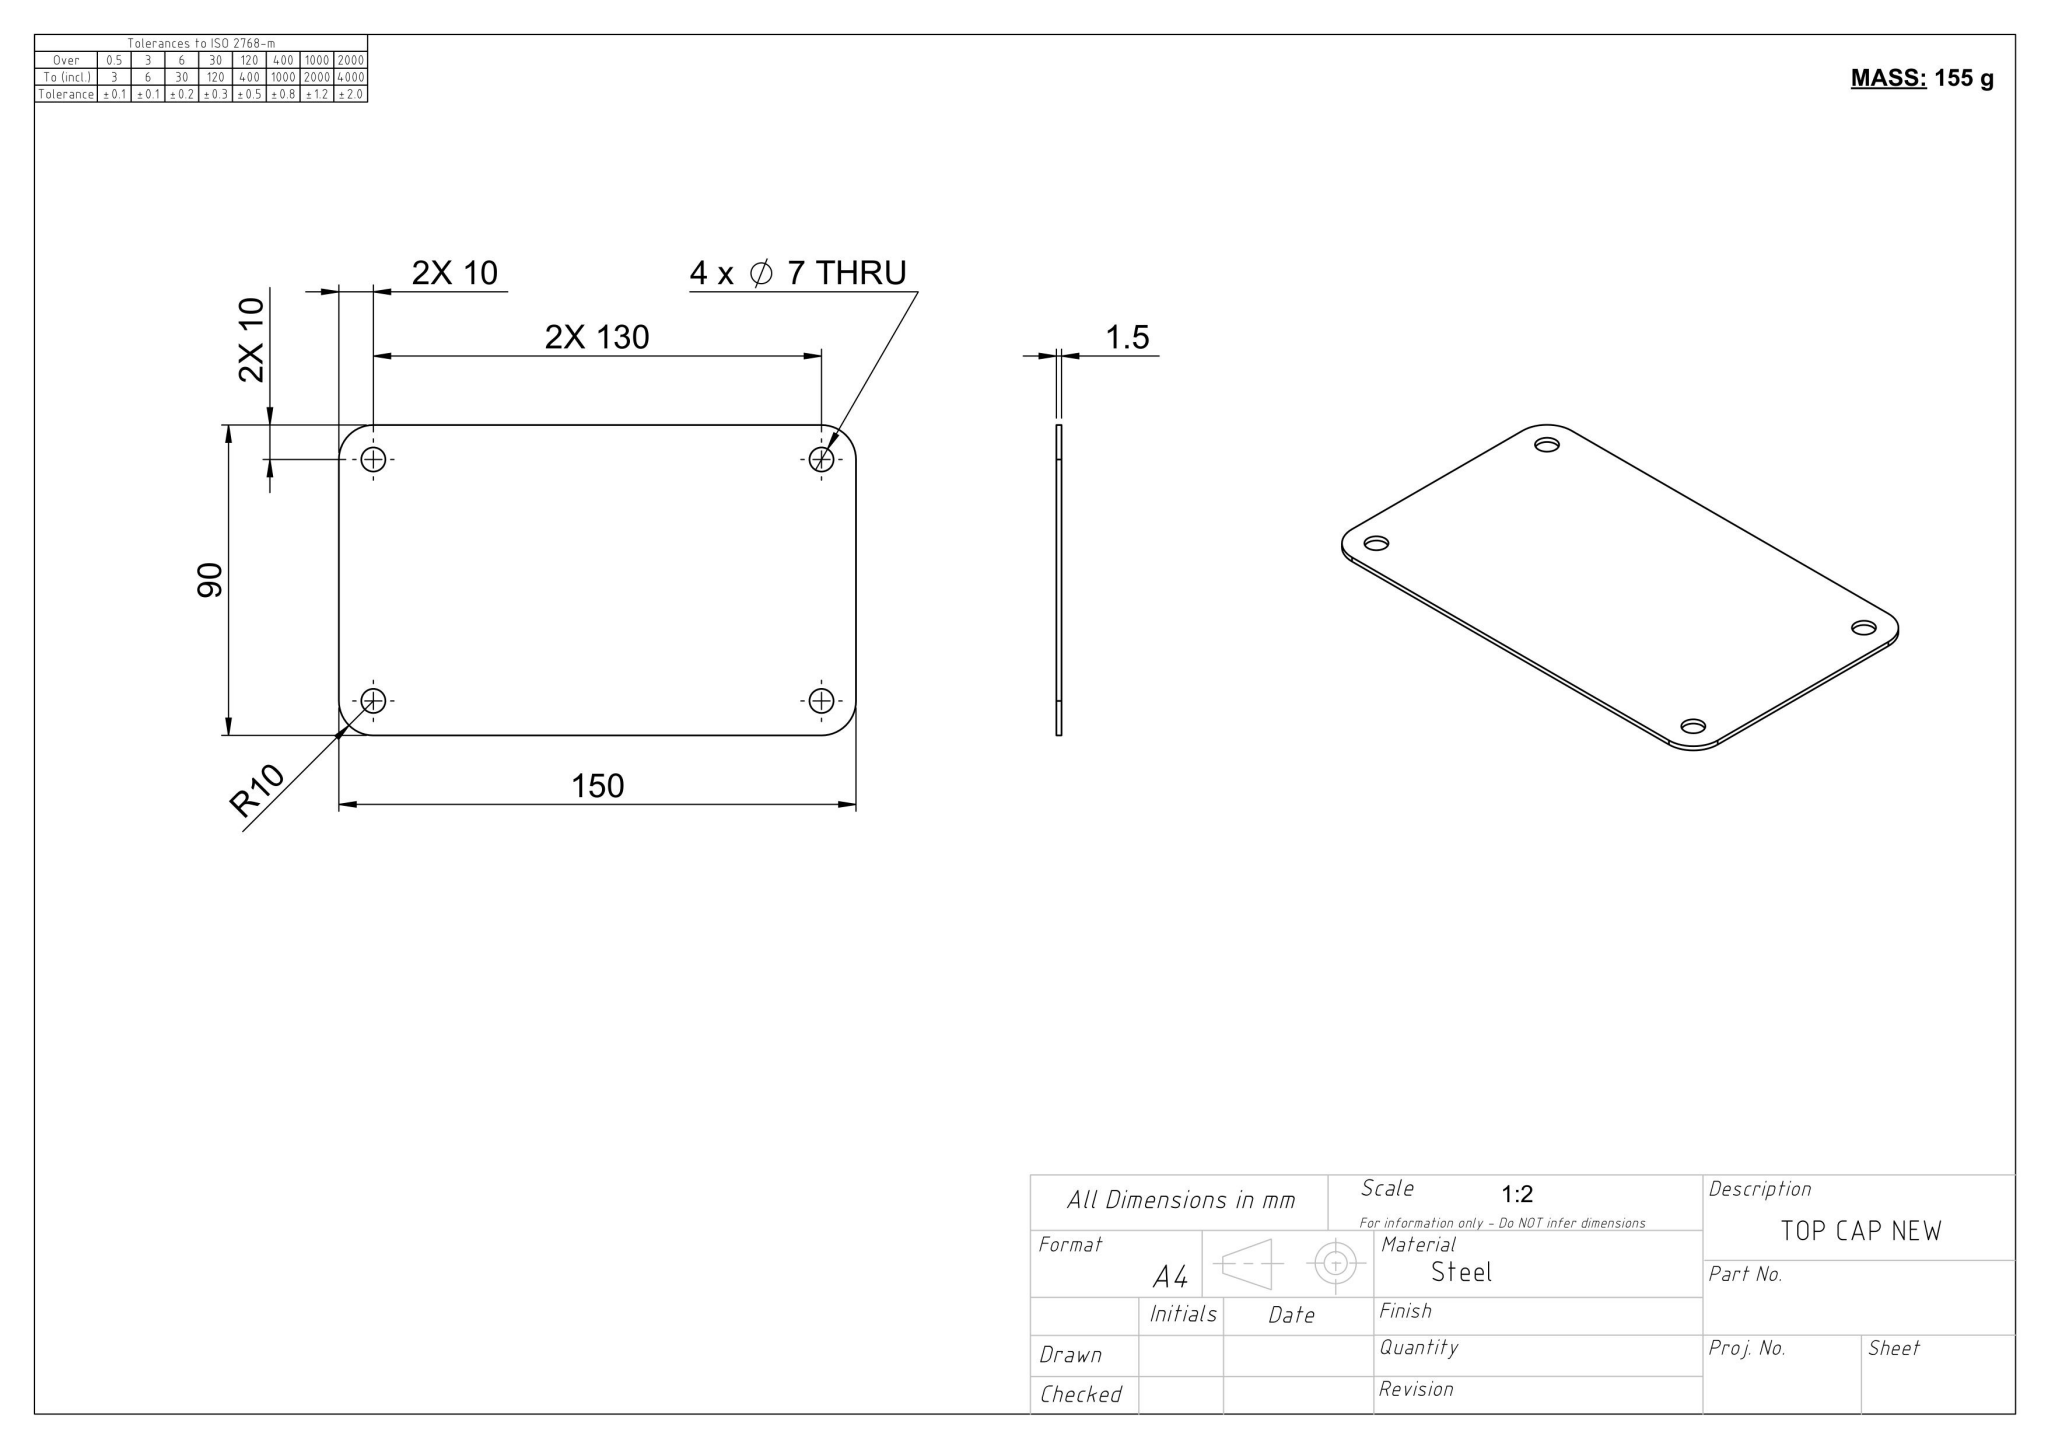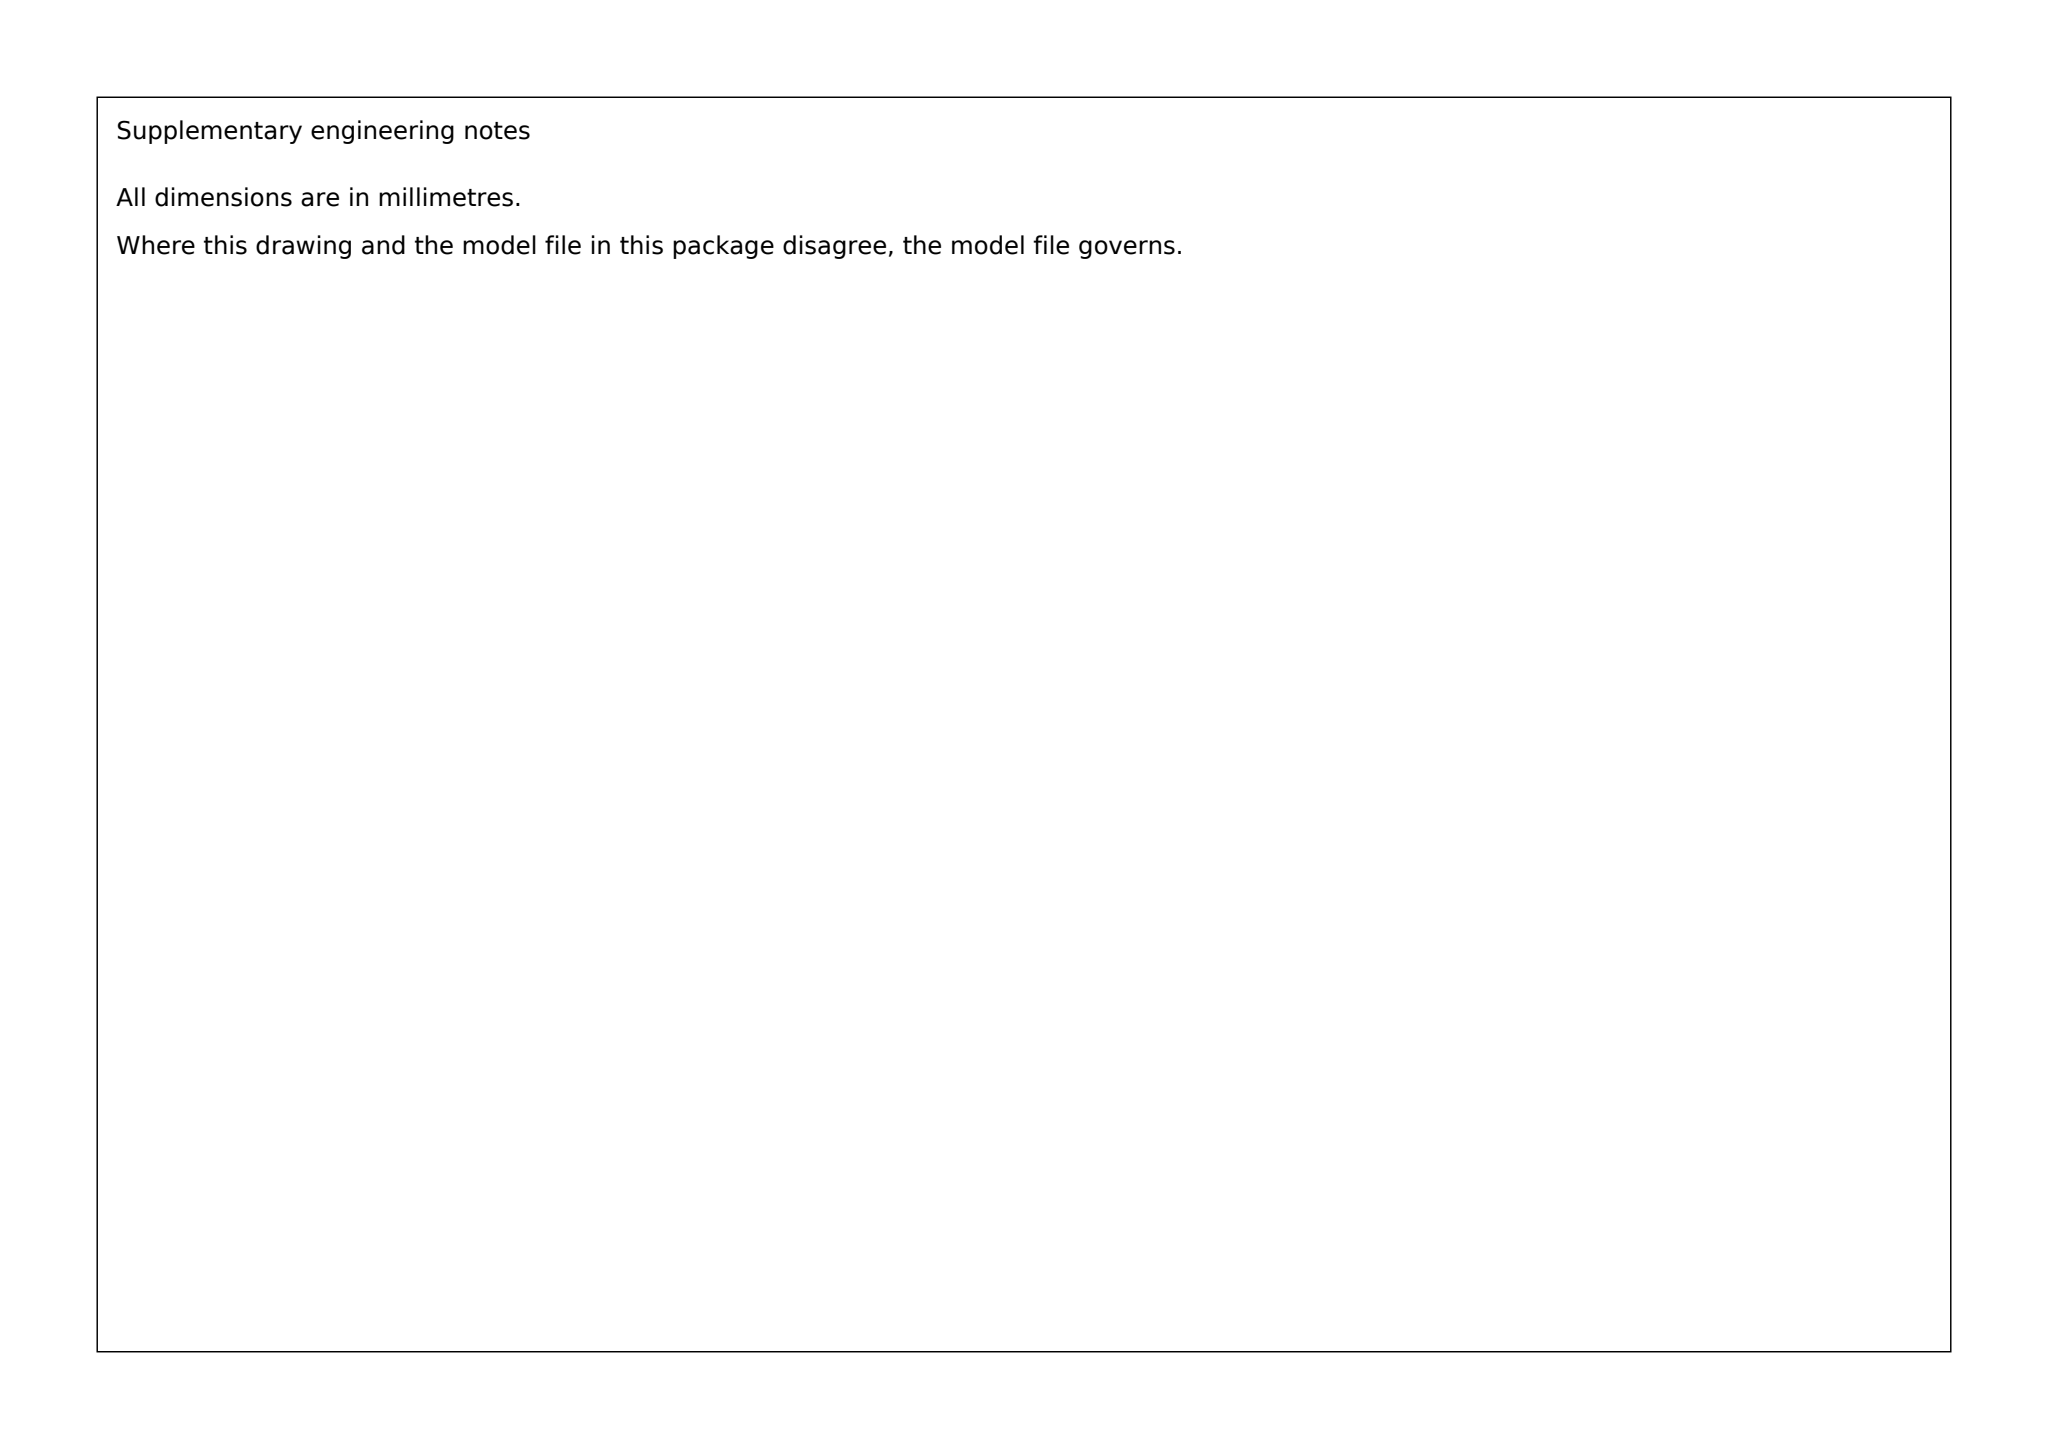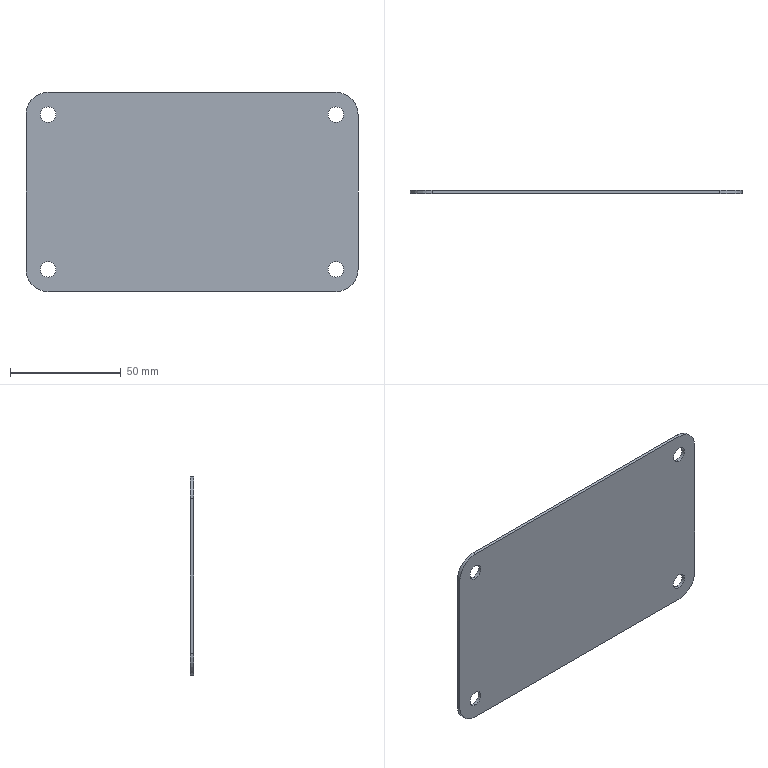Part | SolidWorks | mm | material Steel | 1 solid | 18 faces | box 150 x 1.5 x 90 mm | volume 19890 mm3 | cylinder 12 | plane 6 | commonest cylinder face diameters 7 x8 20 x4
STEP:
#1=CARTESIAN_POINT('',(-65.,0.,-38.5));
#2=VERTEX_POINT('',#1);
#3=CARTESIAN_POINT('',(-65.,0.,-31.5));
#4=VERTEX_POINT('',#3);
#5=CARTESIAN_POINT('',(-65.,0.,-35.));
#6=DIRECTION('',(0.,1.,0.));
#7=DIRECTION('',(0.,0.,1.));
#8=AXIS2_PLACEMENT_3D('',#5,#6,#7);
#9=CIRCLE('',#8,3.5);
#10=EDGE_CURVE('',#2,#4,#9,.T.);
#11=ORIENTED_EDGE('',*,*,#10,.F.);
#12=CARTESIAN_POINT('',(-65.,1.5,-38.5));
#13=VERTEX_POINT('',#12);
#14=CARTESIAN_POINT('',(-65.,1.5,-38.5));
#15=DIRECTION('',(0.,1.,0.));
#16=VECTOR('',#15,1000.);
#17=LINE('',#14,#16);
#18=EDGE_CURVE('',#2,#13,#17,.T.);
#19=ORIENTED_EDGE('',*,*,#18,.T.);
#20=CARTESIAN_POINT('',(-65.,1.5,-31.5));
#21=VERTEX_POINT('',#20);
#22=CARTESIAN_POINT('',(-65.,1.5,-35.));
#23=DIRECTION('',(0.,1.,0.));
#24=DIRECTION('',(0.,0.,1.));
#25=AXIS2_PLACEMENT_3D('',#22,#23,#24);
#26=CIRCLE('',#25,3.5);
#27=EDGE_CURVE('',#13,#21,#26,.T.);
#28=ORIENTED_EDGE('',*,*,#27,.T.);
#29=CARTESIAN_POINT('',(-65.,1.5,-31.5));
#30=DIRECTION('',(0.,1.,0.));
#31=VECTOR('',#30,1000.);
#32=LINE('',#29,#31);
#33=EDGE_CURVE('',#4,#21,#32,.T.);
#34=ORIENTED_EDGE('',*,*,#33,.F.);
#35=EDGE_LOOP('',(#11,#19,#28,#34));
#36=FACE_OUTER_BOUND('',#35,.T.);
#37=CARTESIAN_POINT('',(-65.,1.5,-35.));
#38=DIRECTION('',(0.,1.,0.));
#39=DIRECTION('',(0.,0.,1.));
#40=AXIS2_PLACEMENT_3D('',#37,#38,#39);
#41=CYLINDRICAL_SURFACE('',#40,3.5);
#42=ADVANCED_FACE('',(#36),#41,.F.);
#43=CARTESIAN_POINT('',(65.,0.,-38.5));
#44=VERTEX_POINT('',#43);
#45=CARTESIAN_POINT('',(65.,0.,-31.5));
#46=VERTEX_POINT('',#45);
#47=CARTESIAN_POINT('',(65.,0.,-35.));
#48=DIRECTION('',(0.,1.,0.));
#49=DIRECTION('',(0.,0.,1.));
#50=AXIS2_PLACEMENT_3D('',#47,#48,#49);
#51=CIRCLE('',#50,3.5);
#52=EDGE_CURVE('',#44,#46,#51,.T.);
#53=ORIENTED_EDGE('',*,*,#52,.F.);
#54=CARTESIAN_POINT('',(65.,1.5,-38.5));
#55=VERTEX_POINT('',#54);
#56=CARTESIAN_POINT('',(65.,1.5,-38.5));
#57=DIRECTION('',(0.,1.,0.));
#58=VECTOR('',#57,1000.);
#59=LINE('',#56,#58);
#60=EDGE_CURVE('',#44,#55,#59,.T.);
#61=ORIENTED_EDGE('',*,*,#60,.T.);
#62=CARTESIAN_POINT('',(65.,1.5,-31.5));
#63=VERTEX_POINT('',#62);
#64=CARTESIAN_POINT('',(65.,1.5,-35.));
#65=DIRECTION('',(0.,1.,0.));
#66=DIRECTION('',(0.,0.,1.));
#67=AXIS2_PLACEMENT_3D('',#64,#65,#66);
#68=CIRCLE('',#67,3.5);
#69=EDGE_CURVE('',#55,#63,#68,.T.);
#70=ORIENTED_EDGE('',*,*,#69,.T.);
#71=CARTESIAN_POINT('',(65.,1.5,-31.5));
#72=DIRECTION('',(0.,1.,0.));
#73=VECTOR('',#72,1000.);
#74=LINE('',#71,#73);
#75=EDGE_CURVE('',#46,#63,#74,.T.);
#76=ORIENTED_EDGE('',*,*,#75,.F.);
#77=EDGE_LOOP('',(#53,#61,#70,#76));
#78=FACE_OUTER_BOUND('',#77,.T.);
#79=CARTESIAN_POINT('',(65.,1.5,-35.));
#80=DIRECTION('',(0.,1.,0.));
#81=DIRECTION('',(0.,0.,1.));
#82=AXIS2_PLACEMENT_3D('',#79,#80,#81);
#83=CYLINDRICAL_SURFACE('',#82,3.5);
#84=ADVANCED_FACE('',(#78),#83,.F.);
#85=CARTESIAN_POINT('',(-65.,0.,31.5));
#86=VERTEX_POINT('',#85);
#87=CARTESIAN_POINT('',(-65.,0.,38.5));
#88=VERTEX_POINT('',#87);
#89=CARTESIAN_POINT('',(-65.,0.,35.));
#90=DIRECTION('',(0.,1.,0.));
#91=DIRECTION('',(0.,0.,1.));
#92=AXIS2_PLACEMENT_3D('',#89,#90,#91);
#93=CIRCLE('',#92,3.5);
#94=EDGE_CURVE('',#86,#88,#93,.T.);
#95=ORIENTED_EDGE('',*,*,#94,.F.);
#96=CARTESIAN_POINT('',(-65.,1.5,31.5));
#97=VERTEX_POINT('',#96);
#98=CARTESIAN_POINT('',(-65.,1.5,31.5));
#99=DIRECTION('',(0.,1.,0.));
#100=VECTOR('',#99,1000.);
#101=LINE('',#98,#100);
#102=EDGE_CURVE('',#86,#97,#101,.T.);
#103=ORIENTED_EDGE('',*,*,#102,.T.);
#104=CARTESIAN_POINT('',(-65.,1.5,38.5));
#105=VERTEX_POINT('',#104);
#106=CARTESIAN_POINT('',(-65.,1.5,35.));
#107=DIRECTION('',(0.,1.,0.));
#108=DIRECTION('',(0.,0.,1.));
#109=AXIS2_PLACEMENT_3D('',#106,#107,#108);
#110=CIRCLE('',#109,3.5);
#111=EDGE_CURVE('',#97,#105,#110,.T.);
#112=ORIENTED_EDGE('',*,*,#111,.T.);
#113=CARTESIAN_POINT('',(-65.,1.5,38.5));
#114=DIRECTION('',(0.,1.,0.));
#115=VECTOR('',#114,1000.);
#116=LINE('',#113,#115);
#117=EDGE_CURVE('',#88,#105,#116,.T.);
#118=ORIENTED_EDGE('',*,*,#117,.F.);
#119=EDGE_LOOP('',(#95,#103,#112,#118));
#120=FACE_OUTER_BOUND('',#119,.T.);
#121=CARTESIAN_POINT('',(-65.,1.5,35.));
#122=DIRECTION('',(0.,1.,0.));
#123=DIRECTION('',(0.,0.,1.));
#124=AXIS2_PLACEMENT_3D('',#121,#122,#123);
#125=CYLINDRICAL_SURFACE('',#124,3.5);
#126=ADVANCED_FACE('',(#120),#125,.F.);
#127=CARTESIAN_POINT('',(65.,0.,31.5));
#128=VERTEX_POINT('',#127);
#129=CARTESIAN_POINT('',(65.,0.,38.5));
#130=VERTEX_POINT('',#129);
#131=CARTESIAN_POINT('',(65.,0.,35.));
#132=DIRECTION('',(0.,1.,0.));
#133=DIRECTION('',(0.,0.,1.));
#134=AXIS2_PLACEMENT_3D('',#131,#132,#133);
#135=CIRCLE('',#134,3.5);
#136=EDGE_CURVE('',#128,#130,#135,.T.);
#137=ORIENTED_EDGE('',*,*,#136,.F.);
#138=CARTESIAN_POINT('',(65.,1.5,31.5));
#139=VERTEX_POINT('',#138);
#140=CARTESIAN_POINT('',(65.,1.5,31.5));
#141=DIRECTION('',(0.,1.,0.));
#142=VECTOR('',#141,1000.);
#143=LINE('',#140,#142);
#144=EDGE_CURVE('',#128,#139,#143,.T.);
#145=ORIENTED_EDGE('',*,*,#144,.T.);
#146=CARTESIAN_POINT('',(65.,1.5,38.5));
#147=VERTEX_POINT('',#146);
#148=CARTESIAN_POINT('',(65.,1.5,35.));
#149=DIRECTION('',(0.,1.,0.));
#150=DIRECTION('',(0.,0.,1.));
#151=AXIS2_PLACEMENT_3D('',#148,#149,#150);
#152=CIRCLE('',#151,3.5);
#153=EDGE_CURVE('',#139,#147,#152,.T.);
#154=ORIENTED_EDGE('',*,*,#153,.T.);
#155=CARTESIAN_POINT('',(65.,1.5,38.5));
#156=DIRECTION('',(0.,1.,0.));
#157=VECTOR('',#156,1000.);
#158=LINE('',#155,#157);
#159=EDGE_CURVE('',#130,#147,#158,.T.);
#160=ORIENTED_EDGE('',*,*,#159,.F.);
#161=EDGE_LOOP('',(#137,#145,#154,#160));
#162=FACE_OUTER_BOUND('',#161,.T.);
#163=CARTESIAN_POINT('',(65.,1.5,35.));
#164=DIRECTION('',(0.,1.,0.));
#165=DIRECTION('',(0.,0.,1.));
#166=AXIS2_PLACEMENT_3D('',#163,#164,#165);
#167=CYLINDRICAL_SURFACE('',#166,3.5);
#168=ADVANCED_FACE('',(#162),#167,.F.);
#169=CARTESIAN_POINT('',(75.,1.5,35.));
#170=VERTEX_POINT('',#169);
#171=CARTESIAN_POINT('',(75.,1.5,-35.));
#172=VERTEX_POINT('',#171);
#173=CARTESIAN_POINT('',(75.,1.5,-45.));
#174=DIRECTION('',(0.,0.,-1.));
#175=VECTOR('',#174,1000.);
#176=LINE('',#173,#175);
#177=EDGE_CURVE('',#170,#172,#176,.T.);
#178=ORIENTED_EDGE('',*,*,#177,.F.);
#179=CARTESIAN_POINT('',(75.,0.,35.));
#180=VERTEX_POINT('',#179);
#181=CARTESIAN_POINT('',(75.,1.5,35.));
#182=DIRECTION('',(0.,-1.,0.));
#183=VECTOR('',#182,1000.);
#184=LINE('',#181,#183);
#185=EDGE_CURVE('',#170,#180,#184,.T.);
#186=ORIENTED_EDGE('',*,*,#185,.T.);
#187=CARTESIAN_POINT('',(75.,0.,-35.));
#188=VERTEX_POINT('',#187);
#189=CARTESIAN_POINT('',(75.,0.,-45.));
#190=DIRECTION('',(0.,0.,-1.));
#191=VECTOR('',#190,1000.);
#192=LINE('',#189,#191);
#193=EDGE_CURVE('',#180,#188,#192,.T.);
#194=ORIENTED_EDGE('',*,*,#193,.T.);
#195=CARTESIAN_POINT('',(75.,1.5,-35.));
#196=DIRECTION('',(0.,1.,0.));
#197=VECTOR('',#196,1000.);
#198=LINE('',#195,#197);
#199=EDGE_CURVE('',#188,#172,#198,.T.);
#200=ORIENTED_EDGE('',*,*,#199,.T.);
#201=EDGE_LOOP('',(#178,#186,#194,#200));
#202=FACE_OUTER_BOUND('',#201,.T.);
#203=CARTESIAN_POINT('',(75.,1.5,-45.));
#204=DIRECTION('',(-1.,0.,-0.));
#205=DIRECTION('',(-0.,0.,1.));
#206=AXIS2_PLACEMENT_3D('',#203,#204,#205);
#207=PLANE('',#206);
#208=ADVANCED_FACE('',(#202),#207,.F.);
#209=CARTESIAN_POINT('',(65.,0.,-45.));
#210=VERTEX_POINT('',#209);
#211=CARTESIAN_POINT('',(-65.,0.,-45.));
#212=VERTEX_POINT('',#211);
#213=CARTESIAN_POINT('',(-75.,0.,-45.));
#214=DIRECTION('',(-1.,0.,0.));
#215=VECTOR('',#214,1000.);
#216=LINE('',#213,#215);
#217=EDGE_CURVE('',#210,#212,#216,.T.);
#218=ORIENTED_EDGE('',*,*,#217,.T.);
#219=CARTESIAN_POINT('',(-65.,1.5,-45.));
#220=VERTEX_POINT('',#219);
#221=CARTESIAN_POINT('',(-65.,1.5,-45.));
#222=DIRECTION('',(0.,1.,0.));
#223=VECTOR('',#222,1000.);
#224=LINE('',#221,#223);
#225=EDGE_CURVE('',#212,#220,#224,.T.);
#226=ORIENTED_EDGE('',*,*,#225,.T.);
#227=CARTESIAN_POINT('',(65.,1.5,-45.));
#228=VERTEX_POINT('',#227);
#229=CARTESIAN_POINT('',(-75.,1.5,-45.));
#230=DIRECTION('',(-1.,0.,0.));
#231=VECTOR('',#230,1000.);
#232=LINE('',#229,#231);
#233=EDGE_CURVE('',#228,#220,#232,.T.);
#234=ORIENTED_EDGE('',*,*,#233,.F.);
#235=CARTESIAN_POINT('',(65.,1.5,-45.));
#236=DIRECTION('',(0.,-1.,0.));
#237=VECTOR('',#236,1000.);
#238=LINE('',#235,#237);
#239=EDGE_CURVE('',#228,#210,#238,.T.);
#240=ORIENTED_EDGE('',*,*,#239,.T.);
#241=EDGE_LOOP('',(#218,#226,#234,#240));
#242=FACE_OUTER_BOUND('',#241,.T.);
#243=CARTESIAN_POINT('',(-75.,1.5,-45.));
#244=DIRECTION('',(0.,0.,1.));
#245=DIRECTION('',(1.,0.,0.));
#246=AXIS2_PLACEMENT_3D('',#243,#244,#245);
#247=PLANE('',#246);
#248=ADVANCED_FACE('',(#242),#247,.F.);
#249=CARTESIAN_POINT('',(-75.,0.,-35.));
#250=VERTEX_POINT('',#249);
#251=CARTESIAN_POINT('',(-75.,0.,35.));
#252=VERTEX_POINT('',#251);
#253=CARTESIAN_POINT('',(-75.,0.,-45.));
#254=DIRECTION('',(0.,0.,1.));
#255=VECTOR('',#254,1000.);
#256=LINE('',#253,#255);
#257=EDGE_CURVE('',#250,#252,#256,.T.);
#258=ORIENTED_EDGE('',*,*,#257,.T.);
#259=CARTESIAN_POINT('',(-75.,1.5,35.));
#260=VERTEX_POINT('',#259);
#261=CARTESIAN_POINT('',(-75.,1.5,35.));
#262=DIRECTION('',(0.,1.,0.));
#263=VECTOR('',#262,1000.);
#264=LINE('',#261,#263);
#265=EDGE_CURVE('',#252,#260,#264,.T.);
#266=ORIENTED_EDGE('',*,*,#265,.T.);
#267=CARTESIAN_POINT('',(-75.,1.5,-35.));
#268=VERTEX_POINT('',#267);
#269=CARTESIAN_POINT('',(-75.,1.5,-45.));
#270=DIRECTION('',(0.,0.,1.));
#271=VECTOR('',#270,1000.);
#272=LINE('',#269,#271);
#273=EDGE_CURVE('',#268,#260,#272,.T.);
#274=ORIENTED_EDGE('',*,*,#273,.F.);
#275=CARTESIAN_POINT('',(-75.,1.5,-35.));
#276=DIRECTION('',(0.,-1.,0.));
#277=VECTOR('',#276,1000.);
#278=LINE('',#275,#277);
#279=EDGE_CURVE('',#268,#250,#278,.T.);
#280=ORIENTED_EDGE('',*,*,#279,.T.);
#281=EDGE_LOOP('',(#258,#266,#274,#280));
#282=FACE_OUTER_BOUND('',#281,.T.);
#283=CARTESIAN_POINT('',(-75.,1.5,-45.));
#284=DIRECTION('',(1.,0.,0.));
#285=DIRECTION('',(0.,0.,-1.));
#286=AXIS2_PLACEMENT_3D('',#283,#284,#285);
#287=PLANE('',#286);
#288=ADVANCED_FACE('',(#282),#287,.F.);
#289=CARTESIAN_POINT('',(-65.,0.,45.));
#290=VERTEX_POINT('',#289);
#291=CARTESIAN_POINT('',(65.,0.,45.));
#292=VERTEX_POINT('',#291);
#293=CARTESIAN_POINT('',(-75.,0.,45.));
#294=DIRECTION('',(1.,0.,0.));
#295=VECTOR('',#294,1000.);
#296=LINE('',#293,#295);
#297=EDGE_CURVE('',#290,#292,#296,.T.);
#298=ORIENTED_EDGE('',*,*,#297,.T.);
#299=CARTESIAN_POINT('',(65.,1.5,45.));
#300=VERTEX_POINT('',#299);
#301=CARTESIAN_POINT('',(65.,1.5,45.));
#302=DIRECTION('',(0.,1.,0.));
#303=VECTOR('',#302,1000.);
#304=LINE('',#301,#303);
#305=EDGE_CURVE('',#292,#300,#304,.T.);
#306=ORIENTED_EDGE('',*,*,#305,.T.);
#307=CARTESIAN_POINT('',(-65.,1.5,45.));
#308=VERTEX_POINT('',#307);
#309=CARTESIAN_POINT('',(-75.,1.5,45.));
#310=DIRECTION('',(1.,0.,0.));
#311=VECTOR('',#310,1000.);
#312=LINE('',#309,#311);
#313=EDGE_CURVE('',#308,#300,#312,.T.);
#314=ORIENTED_EDGE('',*,*,#313,.F.);
#315=CARTESIAN_POINT('',(-65.,1.5,45.));
#316=DIRECTION('',(0.,-1.,0.));
#317=VECTOR('',#316,1000.);
#318=LINE('',#315,#317);
#319=EDGE_CURVE('',#308,#290,#318,.T.);
#320=ORIENTED_EDGE('',*,*,#319,.T.);
#321=EDGE_LOOP('',(#298,#306,#314,#320));
#322=FACE_OUTER_BOUND('',#321,.T.);
#323=CARTESIAN_POINT('',(-75.,1.5,45.));
#324=DIRECTION('',(0.,0.,-1.));
#325=DIRECTION('',(-1.,0.,0.));
#326=AXIS2_PLACEMENT_3D('',#323,#324,#325);
#327=PLANE('',#326);
#328=ADVANCED_FACE('',(#322),#327,.F.);
#329=CARTESIAN_POINT('',(-65.,1.5,-35.));
#330=DIRECTION('',(0.,1.,0.));
#331=DIRECTION('',(0.,0.,1.));
#332=AXIS2_PLACEMENT_3D('',#329,#330,#331);
#333=CIRCLE('',#332,3.5);
#334=EDGE_CURVE('',#21,#13,#333,.T.);
#335=ORIENTED_EDGE('',*,*,#334,.F.);
#336=ORIENTED_EDGE('',*,*,#27,.F.);
#337=EDGE_LOOP('',(#335,#336));
#338=FACE_BOUND('',#337,.T.);
#339=CARTESIAN_POINT('',(65.,1.5,-35.));
#340=DIRECTION('',(0.,1.,0.));
#341=DIRECTION('',(0.,0.,1.));
#342=AXIS2_PLACEMENT_3D('',#339,#340,#341);
#343=CIRCLE('',#342,3.5);
#344=EDGE_CURVE('',#63,#55,#343,.T.);
#345=ORIENTED_EDGE('',*,*,#344,.F.);
#346=ORIENTED_EDGE('',*,*,#69,.F.);
#347=EDGE_LOOP('',(#345,#346));
#348=FACE_BOUND('',#347,.T.);
#349=CARTESIAN_POINT('',(-65.,1.5,35.));
#350=DIRECTION('',(0.,1.,0.));
#351=DIRECTION('',(0.,0.,1.));
#352=AXIS2_PLACEMENT_3D('',#349,#350,#351);
#353=CIRCLE('',#352,3.5);
#354=EDGE_CURVE('',#105,#97,#353,.T.);
#355=ORIENTED_EDGE('',*,*,#354,.F.);
#356=ORIENTED_EDGE('',*,*,#111,.F.);
#357=EDGE_LOOP('',(#355,#356));
#358=FACE_BOUND('',#357,.T.);
#359=CARTESIAN_POINT('',(65.,1.5,35.));
#360=DIRECTION('',(0.,1.,0.));
#361=DIRECTION('',(0.,0.,1.));
#362=AXIS2_PLACEMENT_3D('',#359,#360,#361);
#363=CIRCLE('',#362,3.5);
#364=EDGE_CURVE('',#147,#139,#363,.T.);
#365=ORIENTED_EDGE('',*,*,#364,.F.);
#366=ORIENTED_EDGE('',*,*,#153,.F.);
#367=EDGE_LOOP('',(#365,#366));
#368=FACE_BOUND('',#367,.T.);
#369=ORIENTED_EDGE('',*,*,#313,.T.);
#370=CARTESIAN_POINT('',(65.,1.5,35.));
#371=DIRECTION('',(0.,1.,0.));
#372=DIRECTION('',(0.,0.,1.));
#373=AXIS2_PLACEMENT_3D('',#370,#371,#372);
#374=CIRCLE('',#373,10.);
#375=EDGE_CURVE('',#300,#170,#374,.T.);
#376=ORIENTED_EDGE('',*,*,#375,.T.);
#377=ORIENTED_EDGE('',*,*,#177,.T.);
#378=CARTESIAN_POINT('',(65.,1.5,-35.));
#379=DIRECTION('',(0.,1.,0.));
#380=DIRECTION('',(0.,0.,1.));
#381=AXIS2_PLACEMENT_3D('',#378,#379,#380);
#382=CIRCLE('',#381,10.);
#383=EDGE_CURVE('',#172,#228,#382,.T.);
#384=ORIENTED_EDGE('',*,*,#383,.T.);
#385=ORIENTED_EDGE('',*,*,#233,.T.);
#386=CARTESIAN_POINT('',(-65.,1.5,-35.));
#387=DIRECTION('',(0.,1.,0.));
#388=DIRECTION('',(0.,0.,1.));
#389=AXIS2_PLACEMENT_3D('',#386,#387,#388);
#390=CIRCLE('',#389,10.);
#391=EDGE_CURVE('',#220,#268,#390,.T.);
#392=ORIENTED_EDGE('',*,*,#391,.T.);
#393=ORIENTED_EDGE('',*,*,#273,.T.);
#394=CARTESIAN_POINT('',(-65.,1.5,35.));
#395=DIRECTION('',(0.,1.,0.));
#396=DIRECTION('',(0.,0.,1.));
#397=AXIS2_PLACEMENT_3D('',#394,#395,#396);
#398=CIRCLE('',#397,10.);
#399=EDGE_CURVE('',#260,#308,#398,.T.);
#400=ORIENTED_EDGE('',*,*,#399,.T.);
#401=EDGE_LOOP('',(#369,#376,#377,#384,#385,#392,#393,#400));
#402=FACE_OUTER_BOUND('',#401,.T.);
#403=CARTESIAN_POINT('',(0.,1.5,0.));
#404=DIRECTION('',(0.,1.,0.));
#405=DIRECTION('',(0.,0.,1.));
#406=AXIS2_PLACEMENT_3D('',#403,#404,#405);
#407=PLANE('',#406);
#408=ADVANCED_FACE('',(#338,#348,#358,#368,#402),#407,.T.);
#409=CARTESIAN_POINT('',(-65.,0.,-35.));
#410=DIRECTION('',(0.,1.,0.));
#411=DIRECTION('',(0.,0.,1.));
#412=AXIS2_PLACEMENT_3D('',#409,#410,#411);
#413=CIRCLE('',#412,3.5);
#414=EDGE_CURVE('',#4,#2,#413,.T.);
#415=ORIENTED_EDGE('',*,*,#414,.T.);
#416=ORIENTED_EDGE('',*,*,#10,.T.);
#417=EDGE_LOOP('',(#415,#416));
#418=FACE_BOUND('',#417,.T.);
#419=CARTESIAN_POINT('',(65.,0.,-35.));
#420=DIRECTION('',(0.,1.,0.));
#421=DIRECTION('',(0.,0.,1.));
#422=AXIS2_PLACEMENT_3D('',#419,#420,#421);
#423=CIRCLE('',#422,3.5);
#424=EDGE_CURVE('',#46,#44,#423,.T.);
#425=ORIENTED_EDGE('',*,*,#424,.T.);
#426=ORIENTED_EDGE('',*,*,#52,.T.);
#427=EDGE_LOOP('',(#425,#426));
#428=FACE_BOUND('',#427,.T.);
#429=CARTESIAN_POINT('',(-65.,0.,35.));
#430=DIRECTION('',(0.,1.,0.));
#431=DIRECTION('',(0.,0.,1.));
#432=AXIS2_PLACEMENT_3D('',#429,#430,#431);
#433=CIRCLE('',#432,3.5);
#434=EDGE_CURVE('',#88,#86,#433,.T.);
#435=ORIENTED_EDGE('',*,*,#434,.T.);
#436=ORIENTED_EDGE('',*,*,#94,.T.);
#437=EDGE_LOOP('',(#435,#436));
#438=FACE_BOUND('',#437,.T.);
#439=CARTESIAN_POINT('',(65.,0.,35.));
#440=DIRECTION('',(0.,1.,0.));
#441=DIRECTION('',(0.,0.,1.));
#442=AXIS2_PLACEMENT_3D('',#439,#440,#441);
#443=CIRCLE('',#442,3.5);
#444=EDGE_CURVE('',#130,#128,#443,.T.);
#445=ORIENTED_EDGE('',*,*,#444,.T.);
#446=ORIENTED_EDGE('',*,*,#136,.T.);
#447=EDGE_LOOP('',(#445,#446));
#448=FACE_BOUND('',#447,.T.);
#449=ORIENTED_EDGE('',*,*,#193,.F.);
#450=CARTESIAN_POINT('',(65.,0.,35.));
#451=DIRECTION('',(0.,-1.,0.));
#452=DIRECTION('',(0.,0.,1.));
#453=AXIS2_PLACEMENT_3D('',#450,#451,#452);
#454=CIRCLE('',#453,10.);
#455=EDGE_CURVE('',#180,#292,#454,.T.);
#456=ORIENTED_EDGE('',*,*,#455,.T.);
#457=ORIENTED_EDGE('',*,*,#297,.F.);
#458=CARTESIAN_POINT('',(-65.,0.,35.));
#459=DIRECTION('',(0.,-1.,0.));
#460=DIRECTION('',(0.,0.,1.));
#461=AXIS2_PLACEMENT_3D('',#458,#459,#460);
#462=CIRCLE('',#461,10.);
#463=EDGE_CURVE('',#290,#252,#462,.T.);
#464=ORIENTED_EDGE('',*,*,#463,.T.);
#465=ORIENTED_EDGE('',*,*,#257,.F.);
#466=CARTESIAN_POINT('',(-65.,0.,-35.));
#467=DIRECTION('',(0.,-1.,0.));
#468=DIRECTION('',(0.,0.,1.));
#469=AXIS2_PLACEMENT_3D('',#466,#467,#468);
#470=CIRCLE('',#469,10.);
#471=EDGE_CURVE('',#250,#212,#470,.T.);
#472=ORIENTED_EDGE('',*,*,#471,.T.);
#473=ORIENTED_EDGE('',*,*,#217,.F.);
#474=CARTESIAN_POINT('',(65.,0.,-35.));
#475=DIRECTION('',(0.,-1.,0.));
#476=DIRECTION('',(0.,0.,1.));
#477=AXIS2_PLACEMENT_3D('',#474,#475,#476);
#478=CIRCLE('',#477,10.);
#479=EDGE_CURVE('',#210,#188,#478,.T.);
#480=ORIENTED_EDGE('',*,*,#479,.T.);
#481=EDGE_LOOP('',(#449,#456,#457,#464,#465,#472,#473,#480));
#482=FACE_OUTER_BOUND('',#481,.T.);
#483=CARTESIAN_POINT('',(0.,0.,0.));
#484=DIRECTION('',(0.,1.,0.));
#485=DIRECTION('',(0.,0.,1.));
#486=AXIS2_PLACEMENT_3D('',#483,#484,#485);
#487=PLANE('',#486);
#488=ADVANCED_FACE('',(#418,#428,#438,#448,#482),#487,.F.);
#489=ORIENTED_EDGE('',*,*,#375,.F.);
#490=ORIENTED_EDGE('',*,*,#305,.F.);
#491=ORIENTED_EDGE('',*,*,#455,.F.);
#492=ORIENTED_EDGE('',*,*,#185,.F.);
#493=EDGE_LOOP('',(#489,#490,#491,#492));
#494=FACE_OUTER_BOUND('',#493,.T.);
#495=CARTESIAN_POINT('',(65.,1.5,35.));
#496=DIRECTION('',(0.,-1.,0.));
#497=DIRECTION('',(0.,0.,-1.));
#498=AXIS2_PLACEMENT_3D('',#495,#496,#497);
#499=CYLINDRICAL_SURFACE('',#498,10.);
#500=ADVANCED_FACE('',(#494),#499,.T.);
#501=ORIENTED_EDGE('',*,*,#399,.F.);
#502=ORIENTED_EDGE('',*,*,#265,.F.);
#503=ORIENTED_EDGE('',*,*,#463,.F.);
#504=ORIENTED_EDGE('',*,*,#319,.F.);
#505=EDGE_LOOP('',(#501,#502,#503,#504));
#506=FACE_OUTER_BOUND('',#505,.T.);
#507=CARTESIAN_POINT('',(-65.,1.5,35.));
#508=DIRECTION('',(0.,-1.,0.));
#509=DIRECTION('',(0.,0.,-1.));
#510=AXIS2_PLACEMENT_3D('',#507,#508,#509);
#511=CYLINDRICAL_SURFACE('',#510,10.);
#512=ADVANCED_FACE('',(#506),#511,.T.);
#513=ORIENTED_EDGE('',*,*,#391,.F.);
#514=ORIENTED_EDGE('',*,*,#225,.F.);
#515=ORIENTED_EDGE('',*,*,#471,.F.);
#516=ORIENTED_EDGE('',*,*,#279,.F.);
#517=EDGE_LOOP('',(#513,#514,#515,#516));
#518=FACE_OUTER_BOUND('',#517,.T.);
#519=CARTESIAN_POINT('',(-65.,1.5,-35.));
#520=DIRECTION('',(0.,-1.,0.));
#521=DIRECTION('',(0.,0.,-1.));
#522=AXIS2_PLACEMENT_3D('',#519,#520,#521);
#523=CYLINDRICAL_SURFACE('',#522,10.);
#524=ADVANCED_FACE('',(#518),#523,.T.);
#525=ORIENTED_EDGE('',*,*,#383,.F.);
#526=ORIENTED_EDGE('',*,*,#199,.F.);
#527=ORIENTED_EDGE('',*,*,#479,.F.);
#528=ORIENTED_EDGE('',*,*,#239,.F.);
#529=EDGE_LOOP('',(#525,#526,#527,#528));
#530=FACE_OUTER_BOUND('',#529,.T.);
#531=CARTESIAN_POINT('',(65.,1.5,-35.));
#532=DIRECTION('',(0.,-1.,0.));
#533=DIRECTION('',(0.,0.,-1.));
#534=AXIS2_PLACEMENT_3D('',#531,#532,#533);
#535=CYLINDRICAL_SURFACE('',#534,10.);
#536=ADVANCED_FACE('',(#530),#535,.T.);
#537=ORIENTED_EDGE('',*,*,#144,.F.);
#538=ORIENTED_EDGE('',*,*,#444,.F.);
#539=ORIENTED_EDGE('',*,*,#159,.T.);
#540=ORIENTED_EDGE('',*,*,#364,.T.);
#541=EDGE_LOOP('',(#537,#538,#539,#540));
#542=FACE_OUTER_BOUND('',#541,.T.);
#543=CARTESIAN_POINT('',(65.,1.5,35.));
#544=DIRECTION('',(0.,1.,0.));
#545=DIRECTION('',(0.,0.,1.));
#546=AXIS2_PLACEMENT_3D('',#543,#544,#545);
#547=CYLINDRICAL_SURFACE('',#546,3.5);
#548=ADVANCED_FACE('',(#542),#547,.F.);
#549=ORIENTED_EDGE('',*,*,#102,.F.);
#550=ORIENTED_EDGE('',*,*,#434,.F.);
#551=ORIENTED_EDGE('',*,*,#117,.T.);
#552=ORIENTED_EDGE('',*,*,#354,.T.);
#553=EDGE_LOOP('',(#549,#550,#551,#552));
#554=FACE_OUTER_BOUND('',#553,.T.);
#555=CARTESIAN_POINT('',(-65.,1.5,35.));
#556=DIRECTION('',(0.,1.,0.));
#557=DIRECTION('',(0.,0.,1.));
#558=AXIS2_PLACEMENT_3D('',#555,#556,#557);
#559=CYLINDRICAL_SURFACE('',#558,3.5);
#560=ADVANCED_FACE('',(#554),#559,.F.);
#561=ORIENTED_EDGE('',*,*,#60,.F.);
#562=ORIENTED_EDGE('',*,*,#424,.F.);
#563=ORIENTED_EDGE('',*,*,#75,.T.);
#564=ORIENTED_EDGE('',*,*,#344,.T.);
#565=EDGE_LOOP('',(#561,#562,#563,#564));
#566=FACE_OUTER_BOUND('',#565,.T.);
#567=CARTESIAN_POINT('',(65.,1.5,-35.));
#568=DIRECTION('',(0.,1.,0.));
#569=DIRECTION('',(0.,0.,1.));
#570=AXIS2_PLACEMENT_3D('',#567,#568,#569);
#571=CYLINDRICAL_SURFACE('',#570,3.5);
#572=ADVANCED_FACE('',(#566),#571,.F.);
#573=ORIENTED_EDGE('',*,*,#18,.F.);
#574=ORIENTED_EDGE('',*,*,#414,.F.);
#575=ORIENTED_EDGE('',*,*,#33,.T.);
#576=ORIENTED_EDGE('',*,*,#334,.T.);
#577=EDGE_LOOP('',(#573,#574,#575,#576));
#578=FACE_OUTER_BOUND('',#577,.T.);
#579=CARTESIAN_POINT('',(-65.,1.5,-35.));
#580=DIRECTION('',(0.,1.,0.));
#581=DIRECTION('',(0.,0.,1.));
#582=AXIS2_PLACEMENT_3D('',#579,#580,#581);
#583=CYLINDRICAL_SURFACE('',#582,3.5);
#584=ADVANCED_FACE('',(#578),#583,.F.);
#585=CLOSED_SHELL('',(#42,#84,#126,#168,#208,#248,#288,#328,#408,#488,#500,#512,#524,#536,#548,#560,#572,#584));
#586=MANIFOLD_SOLID_BREP('',#585);
#587=CARTESIAN_POINT('',(0.,0.,0.));
#588=DIRECTION('',(0.,0.,1.));
#589=DIRECTION('',(1.,0.,0.));
#590=AXIS2_PLACEMENT_3D('',#587,#588,#589);
#591=(LENGTH_UNIT()NAMED_UNIT(*)SI_UNIT(.MILLI.,.METRE.));
#592=UNCERTAINTY_MEASURE_WITH_UNIT(LENGTH_MEASURE(0.00001),#591,'','');
#593=(NAMED_UNIT(*)PLANE_ANGLE_UNIT()SI_UNIT($,.RADIAN.));
#594=(NAMED_UNIT(*)SI_UNIT($,.STERADIAN.)SOLID_ANGLE_UNIT());
#595=(GEOMETRIC_REPRESENTATION_CONTEXT(3)GLOBAL_UNCERTAINTY_ASSIGNED_CONTEXT((#592))GLOBAL_UNIT_ASSIGNED_CONTEXT((#591,#593,#594))REPRESENTATION_CONTEXT('',''));
#596=ADVANCED_BREP_SHAPE_REPRESENTATION('',(#586,#590),#595);